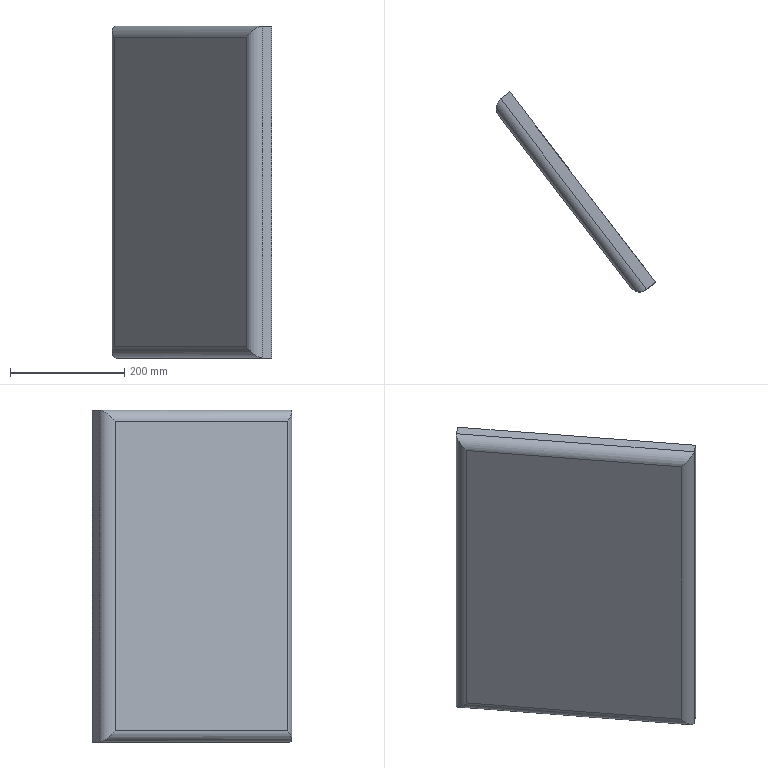Component | NX | GAI | 1 solid | 15 faces | volume 5818758 mm3 | plane 11 | cylinder 4 | commonest cylinder face diameters 40 x4